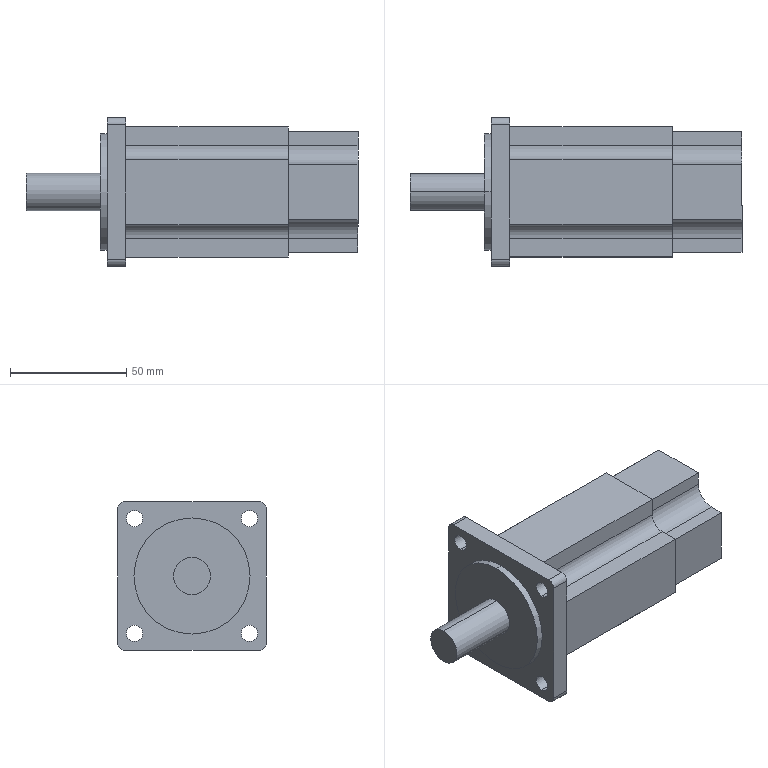Component | SolidWorks | DoubleFilmTransport-1_400WMotor-1 | 1 solid | 58 faces | volume 269850 mm3 | plane 34 | cylinder 24 | commonest cylinder face diameters 7 x8 16 x6 12 x4 6 x4 50 x2